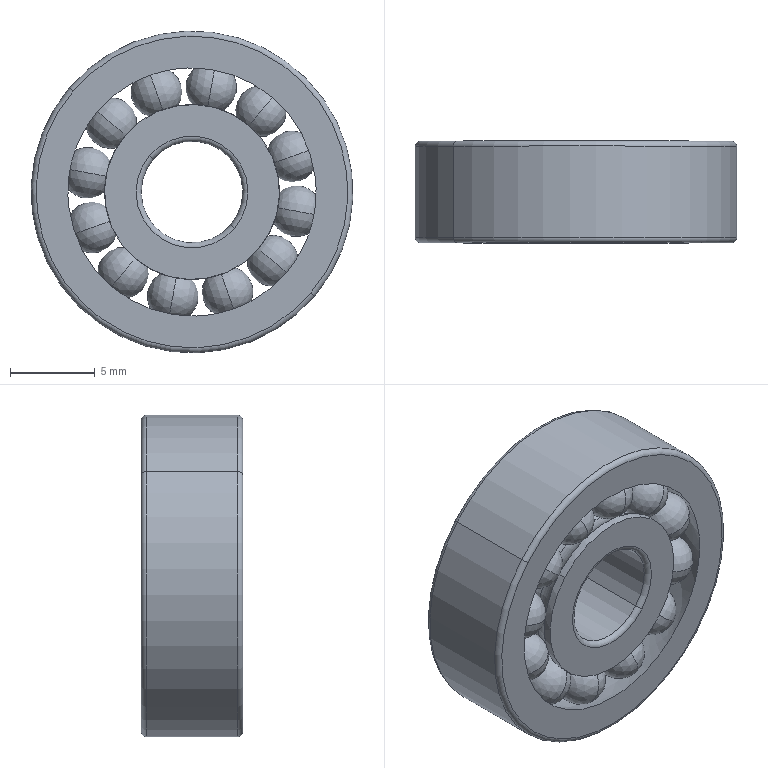Component | SolidWorks | self-aligning ball bearings gb-1 | 1 solid | 120 faces | volume 1210 mm3 | torus 56 | sphere 50 | cylinder 10 | plane 4 | commonest cylinder face diameters 10.333 x6 19 x2 6 x2